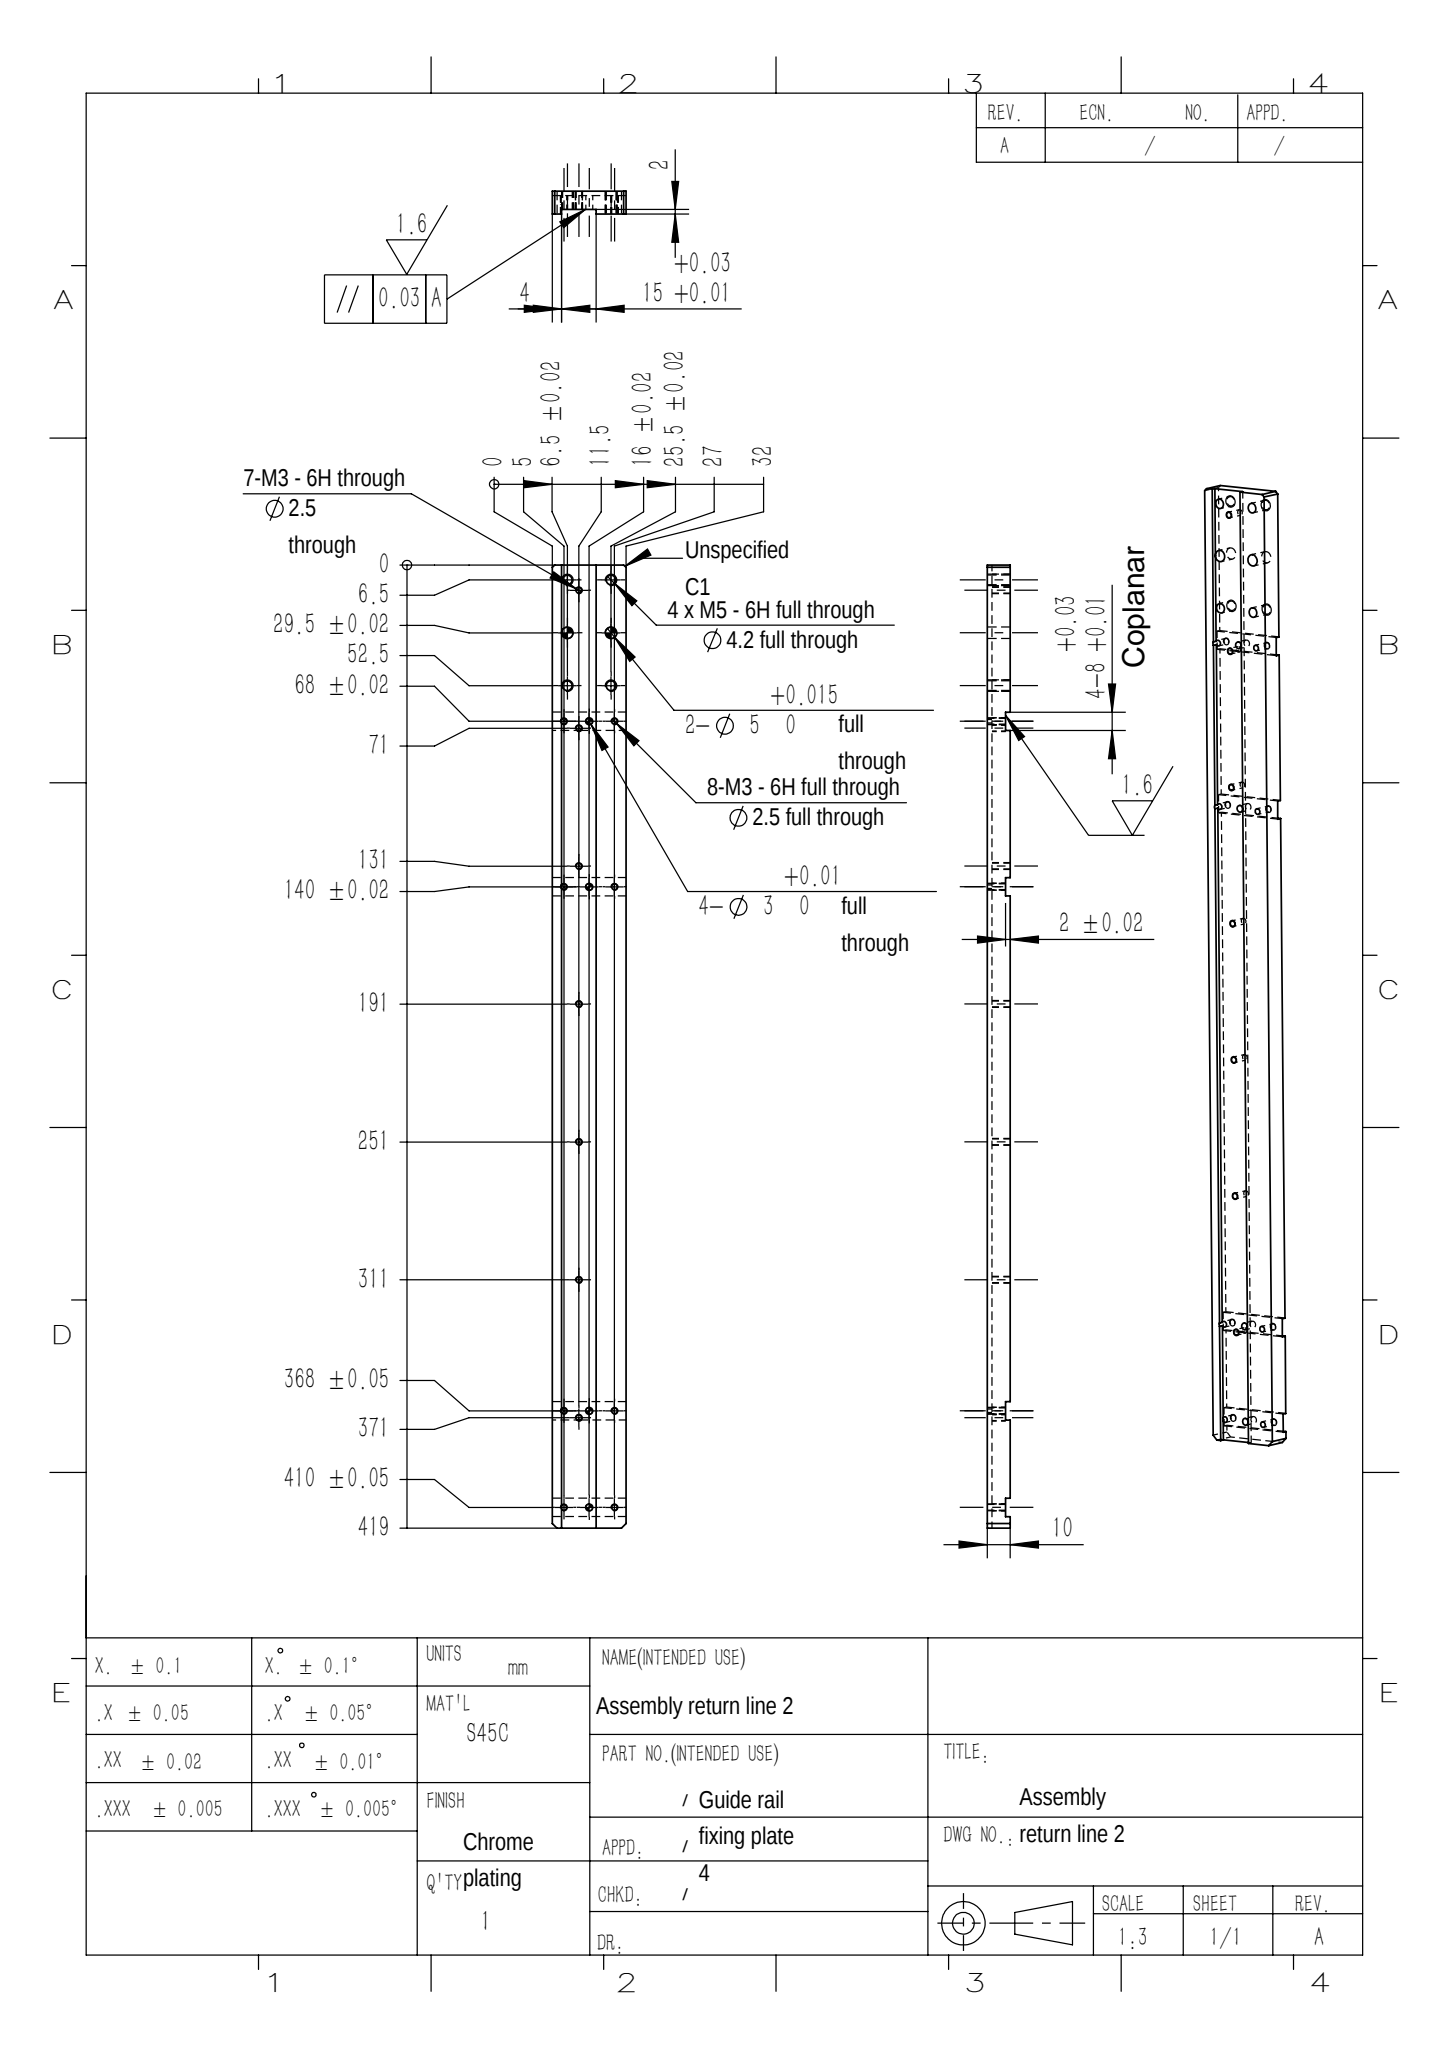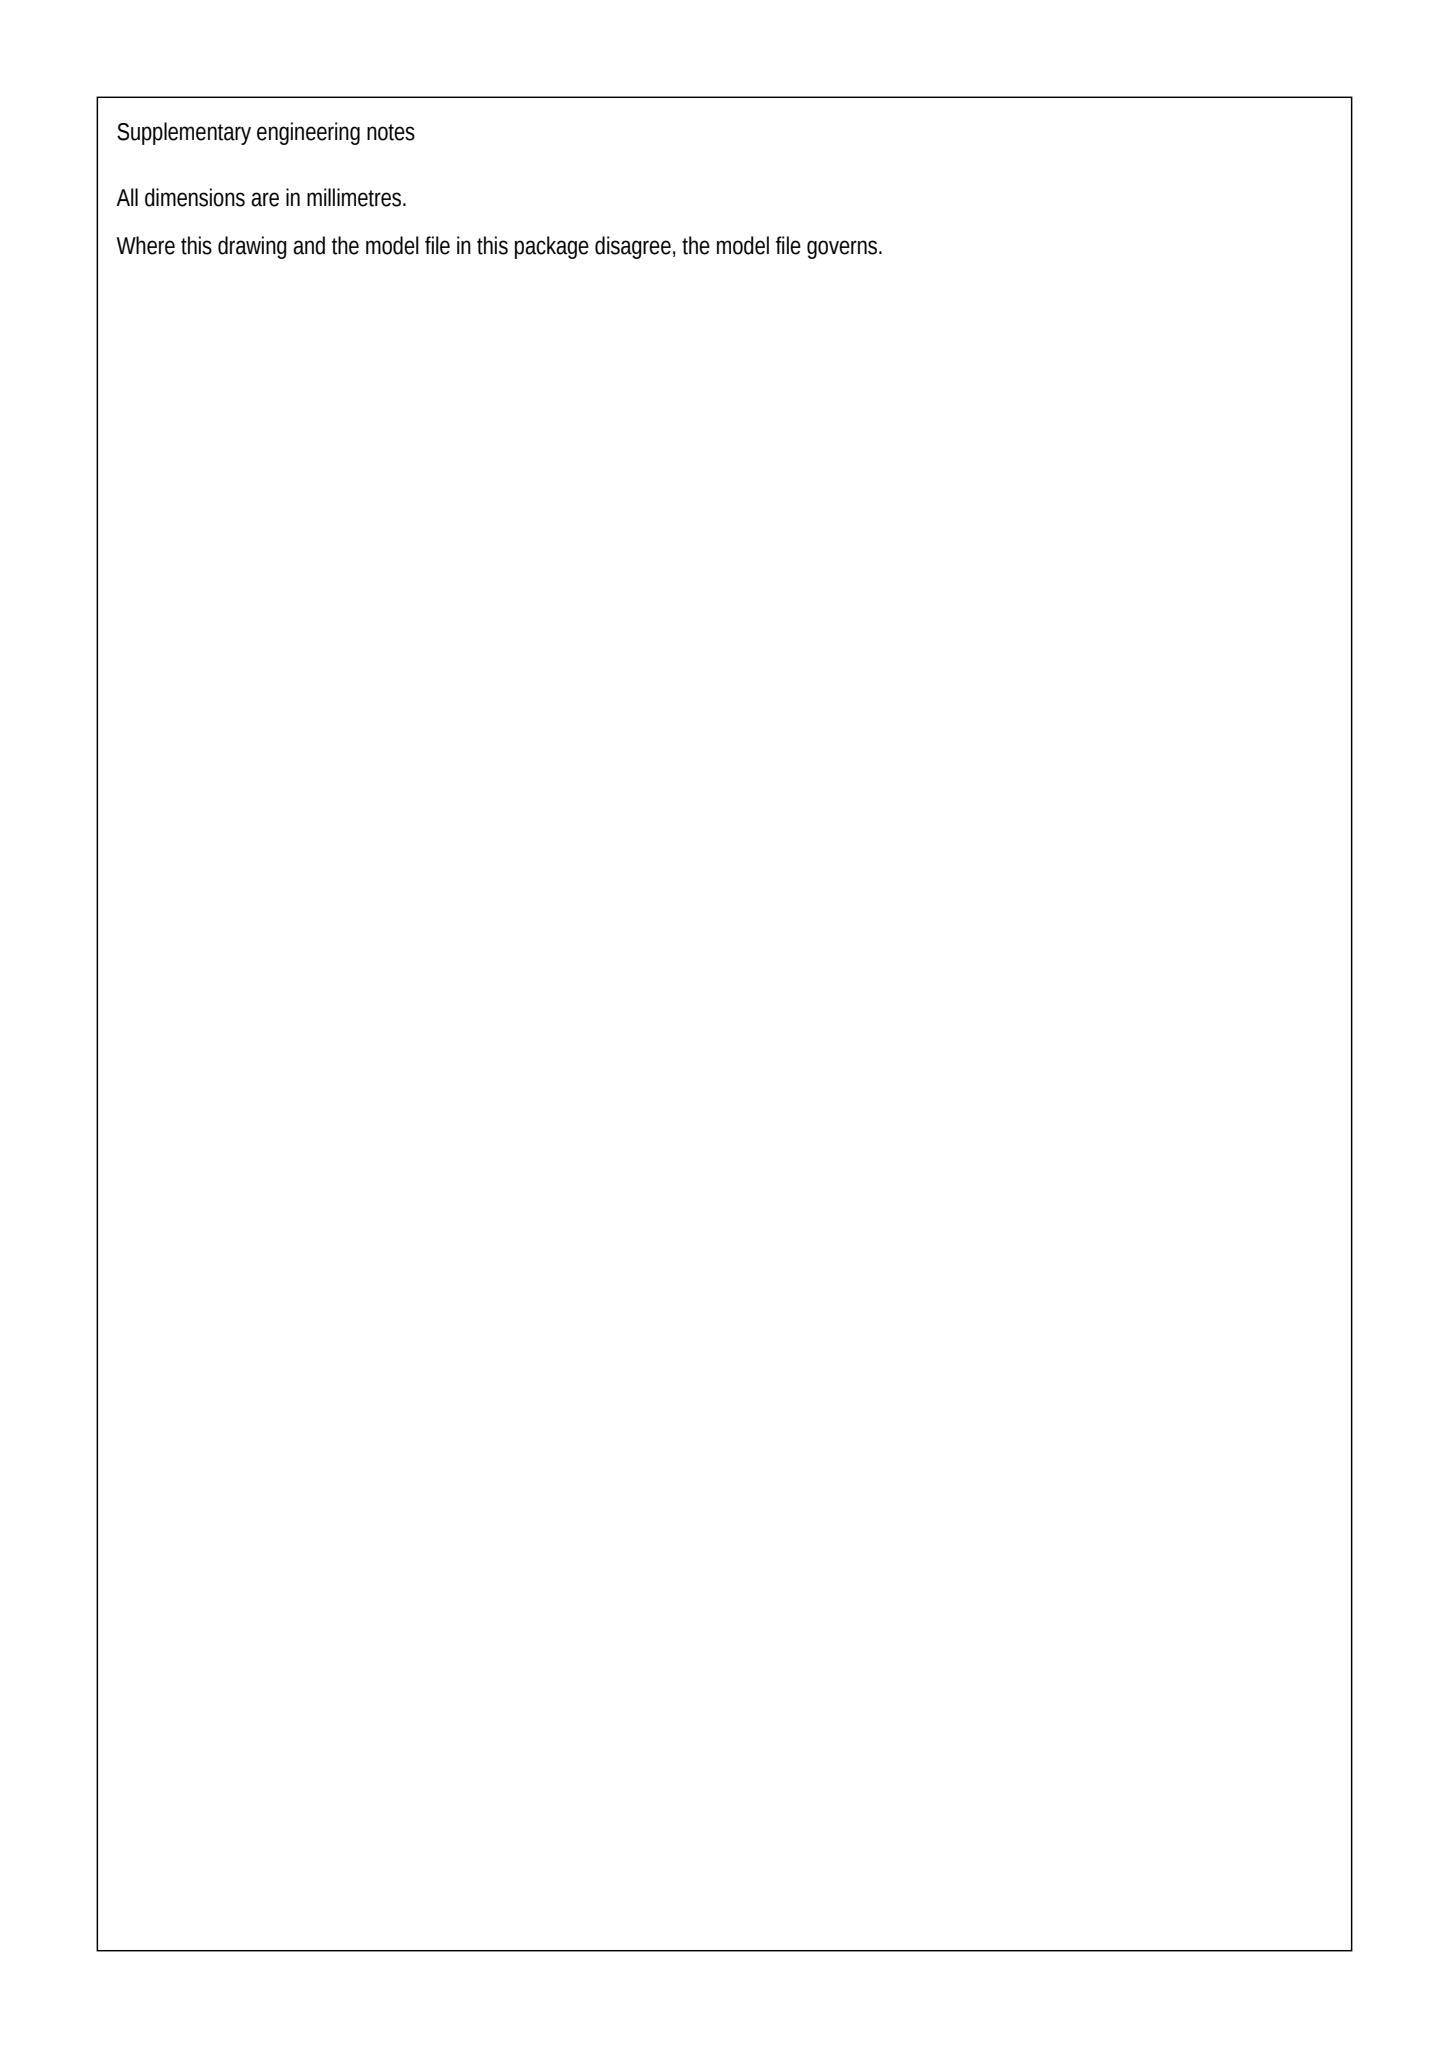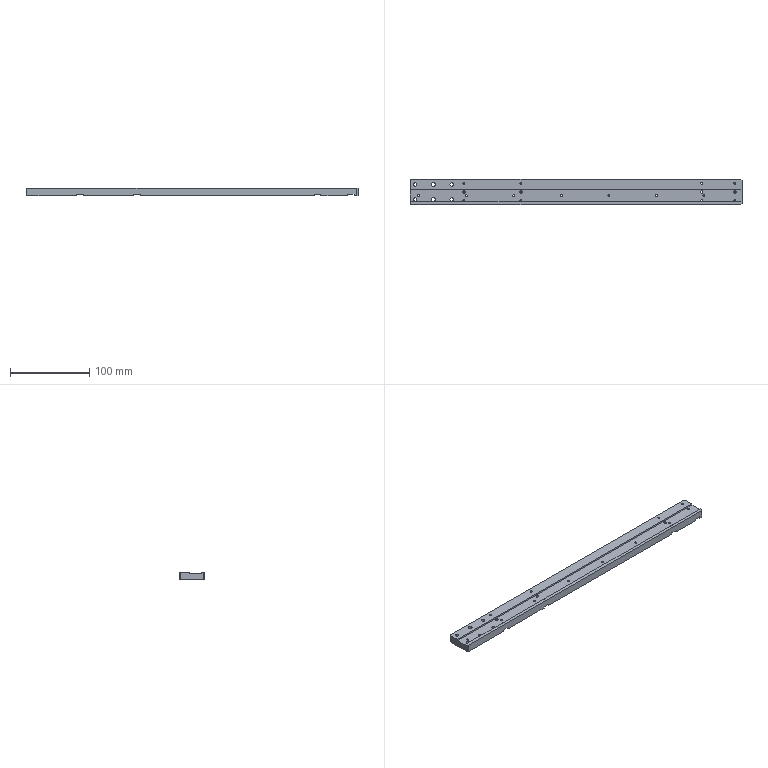Part | SolidWorks | mm | 1 solid | 86 faces | box 419 x 32 x 10 mm | volume 117858 mm3 | cylinder 50 | plane 36 | commonest cylinder face diameters 2.5 x30 4.2 x8 3 x8 5 x4
Drawing notes:
OVERALL 419 X 32 X 10; STEP 19 W X 8 H; RELIEF 4 W X 2 H AT BASE | from the solid: Y planes 0/4/19/32, Z planes 0/2/8/10; bbox 419x32x10
4-8 WIDE RECESS CL AT 68, 140, 368, 410 FROM 0 END, FULL WIDTH 32 | from the solid: X plane pairs 64/72, 136/144, 364/372, 406/414 = 8 wide, centered 68/140/368/410; Z plane 2 floors
M3-6H THRU ON 11.5 CL AT 11 FROM 0 END | from the solid: cylinder Ø2.5 axis z at [11.0, 11.5], length 8.0